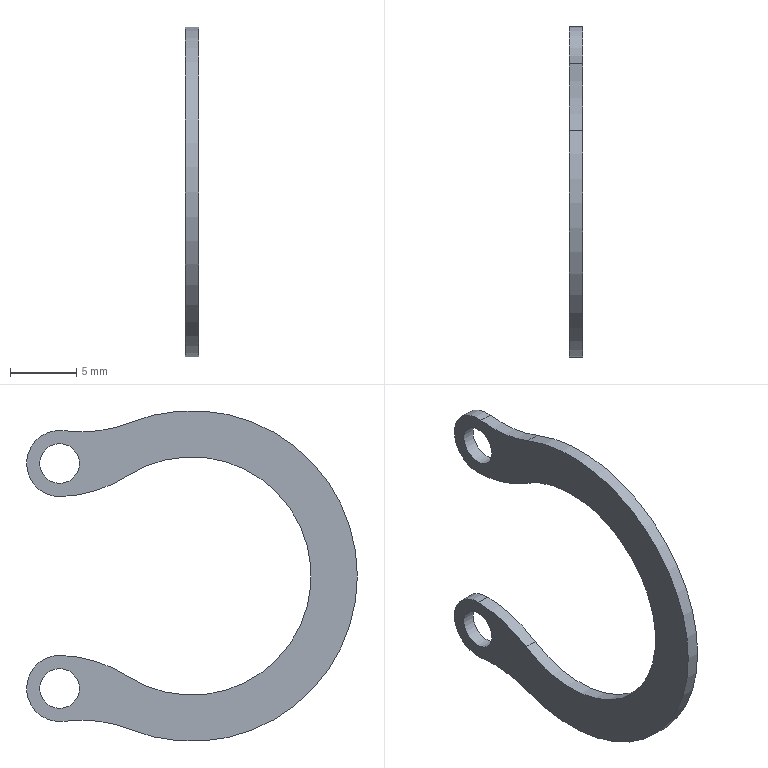Component | NX | SHE_JI-6 | 1 solid | 12 faces | box 1 x 25 x 25 mm | volume 205 mm3 | cylinder 10 | plane 2 | commonest cylinder face diameters 20 x4 5 x2 3 x2 25 x1 18 x1
STEP:
#1=CARTESIAN_POINT('',(0.,0.,0.));
#2=DIRECTION('',(0.,0.,1.));
#3=DIRECTION('',(1.,0.,0.));
#4=AXIS2_PLACEMENT_3D('',#1,#2,#3);
#5=CARTESIAN_POINT('',(85.,29.671,94.022));
#6=VERTEX_POINT('',#5);
#7=CARTESIAN_POINT('',(86.,29.671,94.022));
#8=VERTEX_POINT('',#7);
#9=CARTESIAN_POINT('',(85.,29.671,94.022));
#10=DIRECTION('',(1.,0.,0.));
#11=VECTOR('',#10,1.);
#12=LINE('',#9,#11);
#13=CARTESIAN_POINT('',(85.,28.355,84.109));
#14=DIRECTION('',(1.,0.,0.));
#15=DIRECTION('',(0.,0.,-1.));
#16=AXIS2_PLACEMENT_3D('',#13,#14,#15);
#17=CYLINDRICAL_SURFACE('',#16,10.);
#18=CARTESIAN_POINT('',(3.01,0.));
#19=DIRECTION('',(0.,1.));
#20=VECTOR('',#19,1.);
#21=LINE('',#18,#20);
#22=(GEOMETRIC_REPRESENTATION_CONTEXT(2)PARAMETRIC_REPRESENTATION_CONTEXT()REPRESENTATION_CONTEXT('',''));
#23=DEFINITIONAL_REPRESENTATION('',(#21),#22);
#24=PCURVE('',#17,#23);
#25=CARTESIAN_POINT('',(85.,30.,96.5));
#26=DIRECTION('',(1.,0.,0.));
#27=DIRECTION('',(0.,0.,-1.));
#28=AXIS2_PLACEMENT_3D('',#25,#26,#27);
#29=CYLINDRICAL_SURFACE('',#28,2.5);
#30=CARTESIAN_POINT('',(-0.132,0.));
#31=DIRECTION('',(0.,1.));
#32=VECTOR('',#31,1.);
#33=LINE('',#30,#32);
#34=(GEOMETRIC_REPRESENTATION_CONTEXT(2)PARAMETRIC_REPRESENTATION_CONTEXT()REPRESENTATION_CONTEXT('',''));
#35=DEFINITIONAL_REPRESENTATION('',(#33),#34);
#36=PCURVE('',#29,#35);
#37=SURFACE_CURVE('',#12,(#24,#36),.PCURVE_S1.);
#38=EDGE_CURVE('',#6,#8,#37,.T.);
#39=ORIENTED_EDGE('',*,*,#38,.F.);
#40=CARTESIAN_POINT('',(85.,24.642,93.394));
#41=VERTEX_POINT('',#40);
#42=CARTESIAN_POINT('',(85.,28.355,84.109));
#43=DIRECTION('',(1.,0.,0.));
#44=DIRECTION('',(0.,0.,1.));
#45=AXIS2_PLACEMENT_3D('',#42,#43,#44);
#46=CIRCLE('',#45,10.);
#47=CARTESIAN_POINT('',(-3.142,0.));
#48=DIRECTION('',(1.,0.));
#49=VECTOR('',#48,1.);
#50=LINE('',#47,#49);
#51=(GEOMETRIC_REPRESENTATION_CONTEXT(2)PARAMETRIC_REPRESENTATION_CONTEXT()REPRESENTATION_CONTEXT('',''));
#52=DEFINITIONAL_REPRESENTATION('',(#50),#51);
#53=PCURVE('',#17,#52);
#54=CARTESIAN_POINT('',(85.,24.177,94.554));
#55=DIRECTION('',(1.,0.,0.));
#56=DIRECTION('',(0.,0.,-1.));
#57=AXIS2_PLACEMENT_3D('',#54,#55,#56);
#58=PLANE('',#57);
#59=CARTESIAN_POINT('',(10.446,4.177));
#60=DIRECTION('',(-1.,0.));
#61=AXIS2_PLACEMENT_2D('',#59,#60);
#62=CIRCLE('',#61,10.);
#63=(GEOMETRIC_REPRESENTATION_CONTEXT(2)PARAMETRIC_REPRESENTATION_CONTEXT()REPRESENTATION_CONTEXT('',''));
#64=DEFINITIONAL_REPRESENTATION('',(#62),#63);
#65=PCURVE('',#58,#64);
#66=SURFACE_CURVE('',#46,(#53,#65),.PCURVE_S1.);
#67=EDGE_CURVE('',#6,#41,#66,.T.);
#68=ORIENTED_EDGE('',*,*,#67,.T.);
#69=CARTESIAN_POINT('',(86.,24.642,93.394));
#70=VERTEX_POINT('',#69);
#71=CARTESIAN_POINT('',(85.,24.642,93.394));
#72=DIRECTION('',(1.,0.,0.));
#73=VECTOR('',#72,1.);
#74=LINE('',#71,#73);
#75=CARTESIAN_POINT('',(3.522,0.));
#76=DIRECTION('',(0.,1.));
#77=VECTOR('',#76,1.);
#78=LINE('',#75,#77);
#79=(GEOMETRIC_REPRESENTATION_CONTEXT(2)PARAMETRIC_REPRESENTATION_CONTEXT()REPRESENTATION_CONTEXT('',''));
#80=DEFINITIONAL_REPRESENTATION('',(#78),#79);
#81=PCURVE('',#17,#80);
#82=CARTESIAN_POINT('',(85.,20.,105.));
#83=DIRECTION('',(1.,0.,0.));
#84=DIRECTION('',(0.,0.,-1.));
#85=AXIS2_PLACEMENT_3D('',#82,#83,#84);
#86=CYLINDRICAL_SURFACE('',#85,12.5);
#87=CARTESIAN_POINT('',(6.664,0.));
#88=DIRECTION('',(0.,1.));
#89=VECTOR('',#88,1.);
#90=LINE('',#87,#89);
#91=(GEOMETRIC_REPRESENTATION_CONTEXT(2)PARAMETRIC_REPRESENTATION_CONTEXT()REPRESENTATION_CONTEXT('',''));
#92=DEFINITIONAL_REPRESENTATION('',(#90),#91);
#93=PCURVE('',#86,#92);
#94=SURFACE_CURVE('',#74,(#81,#93),.PCURVE_S1.);
#95=EDGE_CURVE('',#41,#70,#94,.T.);
#96=ORIENTED_EDGE('',*,*,#95,.T.);
#97=CARTESIAN_POINT('',(86.,28.355,84.109));
#98=DIRECTION('',(1.,0.,0.));
#99=DIRECTION('',(0.,0.,1.));
#100=AXIS2_PLACEMENT_3D('',#97,#98,#99);
#101=CIRCLE('',#100,10.);
#102=CARTESIAN_POINT('',(-3.142,1.));
#103=DIRECTION('',(1.,0.));
#104=VECTOR('',#103,1.);
#105=LINE('',#102,#104);
#106=(GEOMETRIC_REPRESENTATION_CONTEXT(2)PARAMETRIC_REPRESENTATION_CONTEXT()REPRESENTATION_CONTEXT('',''));
#107=DEFINITIONAL_REPRESENTATION('',(#105),#106);
#108=PCURVE('',#17,#107);
#109=CARTESIAN_POINT('',(86.,24.177,94.554));
#110=DIRECTION('',(1.,0.,0.));
#111=DIRECTION('',(0.,0.,-1.));
#112=AXIS2_PLACEMENT_3D('',#109,#110,#111);
#113=PLANE('',#112);
#114=CARTESIAN_POINT('',(10.446,4.177));
#115=DIRECTION('',(-1.,0.));
#116=AXIS2_PLACEMENT_2D('',#114,#115);
#117=CIRCLE('',#116,10.);
#118=(GEOMETRIC_REPRESENTATION_CONTEXT(2)PARAMETRIC_REPRESENTATION_CONTEXT()REPRESENTATION_CONTEXT('',''));
#119=DEFINITIONAL_REPRESENTATION('',(#117),#118);
#120=PCURVE('',#113,#119);
#121=SURFACE_CURVE('',#101,(#108,#120),.PCURVE_S1.);
#122=EDGE_CURVE('',#8,#70,#121,.T.);
#123=ORIENTED_EDGE('',*,*,#122,.F.);
#124=EDGE_LOOP('',(#39,#68,#96,#123));
#125=FACE_BOUND('',#124,.F.);
#126=ADVANCED_FACE('',(#125),#17,.F.);
#127=CARTESIAN_POINT('',(86.,24.642,116.606));
#128=VERTEX_POINT('',#127);
#129=CARTESIAN_POINT('',(86.,20.,105.));
#130=DIRECTION('',(-1.,0.,0.));
#131=DIRECTION('',(0.,0.,1.));
#132=AXIS2_PLACEMENT_3D('',#129,#130,#131);
#133=CIRCLE('',#132,12.5);
#134=CARTESIAN_POINT('',(9.425,1.));
#135=DIRECTION('',(-1.,0.));
#136=VECTOR('',#135,1.);
#137=LINE('',#134,#136);
#138=(GEOMETRIC_REPRESENTATION_CONTEXT(2)PARAMETRIC_REPRESENTATION_CONTEXT()REPRESENTATION_CONTEXT('',''));
#139=DEFINITIONAL_REPRESENTATION('',(#137),#138);
#140=PCURVE('',#86,#139);
#141=CARTESIAN_POINT('',(-22.946,-4.177));
#142=CARTESIAN_POINT('',(-22.946,17.473));
#143=CARTESIAN_POINT('',(-4.196,6.648));
#144=CARTESIAN_POINT('',(14.554,-4.177));
#145=CARTESIAN_POINT('',(-4.196,-15.003));
#146=CARTESIAN_POINT('',(-22.946,-25.828));
#147=CARTESIAN_POINT('',(-22.946,-4.177));
#148=(BOUNDED_CURVE()B_SPLINE_CURVE(2,(#141,#142,#143,#144,#145,#146,#147),.UNSPECIFIED.,.T.,.F.)B_SPLINE_CURVE_WITH_KNOTS((1,2,2,2,2,1),(-2.094,0.,2.094,4.189,6.283,8.378),.UNSPECIFIED.)CURVE()GEOMETRIC_REPRESENTATION_ITEM()RATIONAL_B_SPLINE_CURVE((1.,0.5,1.,0.5,1.,0.5,1.))REPRESENTATION_ITEM(''));
#149=(GEOMETRIC_REPRESENTATION_CONTEXT(2)PARAMETRIC_REPRESENTATION_CONTEXT()REPRESENTATION_CONTEXT('',''));
#150=DEFINITIONAL_REPRESENTATION('',(#148),#149);
#151=PCURVE('',#113,#150);
#152=SURFACE_CURVE('',#133,(#140,#151),.PCURVE_S1.);
#153=EDGE_CURVE('',#70,#128,#152,.T.);
#154=ORIENTED_EDGE('',*,*,#153,.T.);
#155=CARTESIAN_POINT('',(85.,24.642,116.606));
#156=VERTEX_POINT('',#155);
#157=CARTESIAN_POINT('',(85.,24.642,116.606));
#158=DIRECTION('',(1.,0.,0.));
#159=VECTOR('',#158,1.);
#160=LINE('',#157,#159);
#161=CARTESIAN_POINT('',(2.761,0.));
#162=DIRECTION('',(0.,1.));
#163=VECTOR('',#162,1.);
#164=LINE('',#161,#163);
#165=(GEOMETRIC_REPRESENTATION_CONTEXT(2)PARAMETRIC_REPRESENTATION_CONTEXT()REPRESENTATION_CONTEXT('',''));
#166=DEFINITIONAL_REPRESENTATION('',(#164),#165);
#167=PCURVE('',#86,#166);
#168=CARTESIAN_POINT('',(85.,28.355,125.891));
#169=DIRECTION('',(1.,0.,0.));
#170=DIRECTION('',(0.,0.,-1.));
#171=AXIS2_PLACEMENT_3D('',#168,#169,#170);
#172=CYLINDRICAL_SURFACE('',#171,10.);
#173=CARTESIAN_POINT('',(5.903,0.));
#174=DIRECTION('',(0.,1.));
#175=VECTOR('',#174,1.);
#176=LINE('',#173,#175);
#177=(GEOMETRIC_REPRESENTATION_CONTEXT(2)PARAMETRIC_REPRESENTATION_CONTEXT()REPRESENTATION_CONTEXT('',''));
#178=DEFINITIONAL_REPRESENTATION('',(#176),#177);
#179=PCURVE('',#172,#178);
#180=SURFACE_CURVE('',#160,(#167,#179),.PCURVE_S1.);
#181=EDGE_CURVE('',#156,#128,#180,.T.);
#182=ORIENTED_EDGE('',*,*,#181,.F.);
#183=CARTESIAN_POINT('',(85.,20.,105.));
#184=DIRECTION('',(-1.,0.,0.));
#185=DIRECTION('',(0.,0.,1.));
#186=AXIS2_PLACEMENT_3D('',#183,#184,#185);
#187=CIRCLE('',#186,12.5);
#188=CARTESIAN_POINT('',(9.425,0.));
#189=DIRECTION('',(-1.,0.));
#190=VECTOR('',#189,1.);
#191=LINE('',#188,#190);
#192=(GEOMETRIC_REPRESENTATION_CONTEXT(2)PARAMETRIC_REPRESENTATION_CONTEXT()REPRESENTATION_CONTEXT('',''));
#193=DEFINITIONAL_REPRESENTATION('',(#191),#192);
#194=PCURVE('',#86,#193);
#195=CARTESIAN_POINT('',(-22.946,-4.177));
#196=CARTESIAN_POINT('',(-22.946,17.473));
#197=CARTESIAN_POINT('',(-4.196,6.648));
#198=CARTESIAN_POINT('',(14.554,-4.177));
#199=CARTESIAN_POINT('',(-4.196,-15.003));
#200=CARTESIAN_POINT('',(-22.946,-25.828));
#201=CARTESIAN_POINT('',(-22.946,-4.177));
#202=(BOUNDED_CURVE()B_SPLINE_CURVE(2,(#195,#196,#197,#198,#199,#200,#201),.UNSPECIFIED.,.T.,.F.)B_SPLINE_CURVE_WITH_KNOTS((1,2,2,2,2,1),(-2.094,0.,2.094,4.189,6.283,8.378),.UNSPECIFIED.)CURVE()GEOMETRIC_REPRESENTATION_ITEM()RATIONAL_B_SPLINE_CURVE((1.,0.5,1.,0.5,1.,0.5,1.))REPRESENTATION_ITEM(''));
#203=(GEOMETRIC_REPRESENTATION_CONTEXT(2)PARAMETRIC_REPRESENTATION_CONTEXT()REPRESENTATION_CONTEXT('',''));
#204=DEFINITIONAL_REPRESENTATION('',(#202),#203);
#205=PCURVE('',#58,#204);
#206=SURFACE_CURVE('',#187,(#194,#205),.PCURVE_S1.);
#207=EDGE_CURVE('',#41,#156,#206,.T.);
#208=ORIENTED_EDGE('',*,*,#207,.F.);
#209=ORIENTED_EDGE('',*,*,#95,.T.);
#210=EDGE_LOOP('',(#154,#182,#208,#209));
#211=FACE_BOUND('',#210,.T.);
#212=ADVANCED_FACE('',(#211),#86,.T.);
#213=ORIENTED_EDGE('',*,*,#181,.F.);
#214=CARTESIAN_POINT('',(85.,29.671,115.978));
#215=VERTEX_POINT('',#214);
#216=CARTESIAN_POINT('',(85.,28.355,125.891));
#217=DIRECTION('',(1.,0.,0.));
#218=DIRECTION('',(0.,0.,-1.));
#219=AXIS2_PLACEMENT_3D('',#216,#217,#218);
#220=CIRCLE('',#219,10.);
#221=CARTESIAN_POINT('',(0.,0.));
#222=DIRECTION('',(1.,0.));
#223=VECTOR('',#222,1.);
#224=LINE('',#221,#223);
#225=(GEOMETRIC_REPRESENTATION_CONTEXT(2)PARAMETRIC_REPRESENTATION_CONTEXT()REPRESENTATION_CONTEXT('',''));
#226=DEFINITIONAL_REPRESENTATION('',(#224),#225);
#227=PCURVE('',#172,#226);
#228=CARTESIAN_POINT('',(-31.337,4.177));
#229=DIRECTION('',(1.,0.));
#230=AXIS2_PLACEMENT_2D('',#228,#229);
#231=CIRCLE('',#230,10.);
#232=(GEOMETRIC_REPRESENTATION_CONTEXT(2)PARAMETRIC_REPRESENTATION_CONTEXT()REPRESENTATION_CONTEXT('',''));
#233=DEFINITIONAL_REPRESENTATION('',(#231),#232);
#234=PCURVE('',#58,#233);
#235=SURFACE_CURVE('',#220,(#227,#234),.PCURVE_S1.);
#236=EDGE_CURVE('',#156,#215,#235,.T.);
#237=ORIENTED_EDGE('',*,*,#236,.T.);
#238=CARTESIAN_POINT('',(86.,29.671,115.978));
#239=VERTEX_POINT('',#238);
#240=CARTESIAN_POINT('',(85.,29.671,115.978));
#241=DIRECTION('',(1.,0.,0.));
#242=VECTOR('',#241,1.);
#243=LINE('',#240,#242);
#244=CARTESIAN_POINT('',(6.415,0.));
#245=DIRECTION('',(0.,1.));
#246=VECTOR('',#245,1.);
#247=LINE('',#244,#246);
#248=(GEOMETRIC_REPRESENTATION_CONTEXT(2)PARAMETRIC_REPRESENTATION_CONTEXT()REPRESENTATION_CONTEXT('',''));
#249=DEFINITIONAL_REPRESENTATION('',(#247),#248);
#250=PCURVE('',#172,#249);
#251=CARTESIAN_POINT('',(85.,30.,113.5));
#252=DIRECTION('',(1.,0.,0.));
#253=DIRECTION('',(0.,0.,-1.));
#254=AXIS2_PLACEMENT_3D('',#251,#252,#253);
#255=CYLINDRICAL_SURFACE('',#254,2.5);
#256=CARTESIAN_POINT('',(3.274,0.));
#257=DIRECTION('',(0.,1.));
#258=VECTOR('',#257,1.);
#259=LINE('',#256,#258);
#260=(GEOMETRIC_REPRESENTATION_CONTEXT(2)PARAMETRIC_REPRESENTATION_CONTEXT()REPRESENTATION_CONTEXT('',''));
#261=DEFINITIONAL_REPRESENTATION('',(#259),#260);
#262=PCURVE('',#255,#261);
#263=SURFACE_CURVE('',#243,(#250,#262),.PCURVE_S1.);
#264=EDGE_CURVE('',#215,#239,#263,.T.);
#265=ORIENTED_EDGE('',*,*,#264,.T.);
#266=CARTESIAN_POINT('',(86.,28.355,125.891));
#267=DIRECTION('',(1.,0.,0.));
#268=DIRECTION('',(0.,0.,-1.));
#269=AXIS2_PLACEMENT_3D('',#266,#267,#268);
#270=CIRCLE('',#269,10.);
#271=CARTESIAN_POINT('',(0.,1.));
#272=DIRECTION('',(1.,0.));
#273=VECTOR('',#272,1.);
#274=LINE('',#271,#273);
#275=(GEOMETRIC_REPRESENTATION_CONTEXT(2)PARAMETRIC_REPRESENTATION_CONTEXT()REPRESENTATION_CONTEXT('',''));
#276=DEFINITIONAL_REPRESENTATION('',(#274),#275);
#277=PCURVE('',#172,#276);
#278=CARTESIAN_POINT('',(-31.337,4.177));
#279=DIRECTION('',(1.,0.));
#280=AXIS2_PLACEMENT_2D('',#278,#279);
#281=CIRCLE('',#280,10.);
#282=(GEOMETRIC_REPRESENTATION_CONTEXT(2)PARAMETRIC_REPRESENTATION_CONTEXT()REPRESENTATION_CONTEXT('',''));
#283=DEFINITIONAL_REPRESENTATION('',(#281),#282);
#284=PCURVE('',#113,#283);
#285=SURFACE_CURVE('',#270,(#277,#284),.PCURVE_S1.);
#286=EDGE_CURVE('',#128,#239,#285,.T.);
#287=ORIENTED_EDGE('',*,*,#286,.F.);
#288=EDGE_LOOP('',(#213,#237,#265,#287));
#289=FACE_BOUND('',#288,.F.);
#290=ADVANCED_FACE('',(#289),#172,.F.);
#291=CARTESIAN_POINT('',(86.,29.915,111.001));
#292=VERTEX_POINT('',#291);
#293=CARTESIAN_POINT('',(86.,30.,113.5));
#294=DIRECTION('',(-1.,0.,0.));
#295=DIRECTION('',(0.,0.,-1.));
#296=AXIS2_PLACEMENT_3D('',#293,#294,#295);
#297=CIRCLE('',#296,2.5);
#298=CARTESIAN_POINT('',(6.283,1.));
#299=DIRECTION('',(-1.,0.));
#300=VECTOR('',#299,1.);
#301=LINE('',#298,#300);
#302=(GEOMETRIC_REPRESENTATION_CONTEXT(2)PARAMETRIC_REPRESENTATION_CONTEXT()REPRESENTATION_CONTEXT('',''));
#303=DEFINITIONAL_REPRESENTATION('',(#301),#302);
#304=PCURVE('',#255,#303);
#305=CARTESIAN_POINT('',(-16.446,5.823));
#306=CARTESIAN_POINT('',(-16.446,1.492));
#307=CARTESIAN_POINT('',(-20.196,3.657));
#308=CARTESIAN_POINT('',(-23.946,5.823));
#309=CARTESIAN_POINT('',(-20.196,7.988));
#310=CARTESIAN_POINT('',(-16.446,10.153));
#311=CARTESIAN_POINT('',(-16.446,5.823));
#312=(BOUNDED_CURVE()B_SPLINE_CURVE(2,(#305,#306,#307,#308,#309,#310,#311),.UNSPECIFIED.,.T.,.F.)B_SPLINE_CURVE_WITH_KNOTS((1,2,2,2,2,1),(-2.094,0.,2.094,4.189,6.283,8.378),.UNSPECIFIED.)CURVE()GEOMETRIC_REPRESENTATION_ITEM()RATIONAL_B_SPLINE_CURVE((1.,0.5,1.,0.5,1.,0.5,1.))REPRESENTATION_ITEM(''));
#313=(GEOMETRIC_REPRESENTATION_CONTEXT(2)PARAMETRIC_REPRESENTATION_CONTEXT()REPRESENTATION_CONTEXT('',''));
#314=DEFINITIONAL_REPRESENTATION('',(#312),#313);
#315=PCURVE('',#113,#314);
#316=SURFACE_CURVE('',#297,(#304,#315),.PCURVE_S1.);
#317=EDGE_CURVE('',#239,#292,#316,.T.);
#318=ORIENTED_EDGE('',*,*,#317,.T.);
#319=CARTESIAN_POINT('',(85.,29.915,111.001));
#320=VERTEX_POINT('',#319);
#321=CARTESIAN_POINT('',(85.,29.915,111.001));
#322=DIRECTION('',(1.,0.,0.));
#323=VECTOR('',#322,1.);
#324=LINE('',#321,#323);
#325=CARTESIAN_POINT('',(-0.03383,0.));
#326=DIRECTION('',(0.,1.));
#327=VECTOR('',#326,1.);
#328=LINE('',#325,#327);
#329=(GEOMETRIC_REPRESENTATION_CONTEXT(2)PARAMETRIC_REPRESENTATION_CONTEXT()REPRESENTATION_CONTEXT('',''));
#330=DEFINITIONAL_REPRESENTATION('',(#328),#329);
#331=PCURVE('',#255,#330);
#332=CARTESIAN_POINT('',(85.,30.254,120.996));
#333=DIRECTION('',(1.,0.,0.));
#334=DIRECTION('',(0.,0.,-1.));
#335=AXIS2_PLACEMENT_3D('',#332,#333,#334);
#336=CYLINDRICAL_SURFACE('',#335,10.);
#337=CARTESIAN_POINT('',(6.249,0.));
#338=DIRECTION('',(0.,1.));
#339=VECTOR('',#338,1.);
#340=LINE('',#337,#339);
#341=(GEOMETRIC_REPRESENTATION_CONTEXT(2)PARAMETRIC_REPRESENTATION_CONTEXT()REPRESENTATION_CONTEXT('',''));
#342=DEFINITIONAL_REPRESENTATION('',(#340),#341);
#343=PCURVE('',#336,#342);
#344=SURFACE_CURVE('',#324,(#331,#343),.PCURVE_S1.);
#345=EDGE_CURVE('',#320,#292,#344,.T.);
#346=ORIENTED_EDGE('',*,*,#345,.F.);
#347=CARTESIAN_POINT('',(85.,30.,113.5));
#348=DIRECTION('',(-1.,0.,0.));
#349=DIRECTION('',(0.,0.,-1.));
#350=AXIS2_PLACEMENT_3D('',#347,#348,#349);
#351=CIRCLE('',#350,2.5);
#352=CARTESIAN_POINT('',(6.283,0.));
#353=DIRECTION('',(-1.,0.));
#354=VECTOR('',#353,1.);
#355=LINE('',#352,#354);
#356=(GEOMETRIC_REPRESENTATION_CONTEXT(2)PARAMETRIC_REPRESENTATION_CONTEXT()REPRESENTATION_CONTEXT('',''));
#357=DEFINITIONAL_REPRESENTATION('',(#355),#356);
#358=PCURVE('',#255,#357);
#359=CARTESIAN_POINT('',(-16.446,5.823));
#360=CARTESIAN_POINT('',(-16.446,1.492));
#361=CARTESIAN_POINT('',(-20.196,3.657));
#362=CARTESIAN_POINT('',(-23.946,5.823));
#363=CARTESIAN_POINT('',(-20.196,7.988));
#364=CARTESIAN_POINT('',(-16.446,10.153));
#365=CARTESIAN_POINT('',(-16.446,5.823));
#366=(BOUNDED_CURVE()B_SPLINE_CURVE(2,(#359,#360,#361,#362,#363,#364,#365),.UNSPECIFIED.,.T.,.F.)B_SPLINE_CURVE_WITH_KNOTS((1,2,2,2,2,1),(-2.094,0.,2.094,4.189,6.283,8.378),.UNSPECIFIED.)CURVE()GEOMETRIC_REPRESENTATION_ITEM()RATIONAL_B_SPLINE_CURVE((1.,0.5,1.,0.5,1.,0.5,1.))REPRESENTATION_ITEM(''));
#367=(GEOMETRIC_REPRESENTATION_CONTEXT(2)PARAMETRIC_REPRESENTATION_CONTEXT()REPRESENTATION_CONTEXT('',''));
#368=DEFINITIONAL_REPRESENTATION('',(#366),#367);
#369=PCURVE('',#58,#368);
#370=SURFACE_CURVE('',#351,(#358,#369),.PCURVE_S1.);
#371=EDGE_CURVE('',#215,#320,#370,.T.);
#372=ORIENTED_EDGE('',*,*,#371,.F.);
#373=ORIENTED_EDGE('',*,*,#264,.T.);
#374=EDGE_LOOP('',(#318,#346,#372,#373));
#375=FACE_BOUND('',#374,.T.);
#376=ADVANCED_FACE('',(#375),#255,.T.);
#377=CARTESIAN_POINT('',(86.,24.857,112.577));
#378=VERTEX_POINT('',#377);
#379=CARTESIAN_POINT('',(86.,30.254,120.996));
#380=DIRECTION('',(-1.,0.,0.));
#381=DIRECTION('',(0.,0.,-1.));
#382=AXIS2_PLACEMENT_3D('',#379,#380,#381);
#383=CIRCLE('',#382,10.);
#384=CARTESIAN_POINT('',(6.283,1.));
#385=DIRECTION('',(-1.,0.));
#386=VECTOR('',#385,1.);
#387=LINE('',#384,#386);
#388=(GEOMETRIC_REPRESENTATION_CONTEXT(2)PARAMETRIC_REPRESENTATION_CONTEXT()REPRESENTATION_CONTEXT('',''));
#389=DEFINITIONAL_REPRESENTATION('',(#387),#388);
#390=PCURVE('',#336,#389);
#391=CARTESIAN_POINT('',(-16.441,6.076));
#392=CARTESIAN_POINT('',(-16.441,-11.244));
#393=CARTESIAN_POINT('',(-31.441,-2.584));
#394=CARTESIAN_POINT('',(-46.441,6.076));
#395=CARTESIAN_POINT('',(-31.441,14.736));
#396=CARTESIAN_POINT('',(-16.441,23.397));
#397=CARTESIAN_POINT('',(-16.441,6.076));
#398=(BOUNDED_CURVE()B_SPLINE_CURVE(2,(#391,#392,#393,#394,#395,#396,#397),.UNSPECIFIED.,.T.,.F.)B_SPLINE_CURVE_WITH_KNOTS((1,2,2,2,2,1),(-2.094,0.,2.094,4.189,6.283,8.378),.UNSPECIFIED.)CURVE()GEOMETRIC_REPRESENTATION_ITEM()RATIONAL_B_SPLINE_CURVE((1.,0.5,1.,0.5,1.,0.5,1.))REPRESENTATION_ITEM(''));
#399=(GEOMETRIC_REPRESENTATION_CONTEXT(2)PARAMETRIC_REPRESENTATION_CONTEXT()REPRESENTATION_CONTEXT('',''));
#400=DEFINITIONAL_REPRESENTATION('',(#398),#399);
#401=PCURVE('',#113,#400);
#402=SURFACE_CURVE('',#383,(#390,#401),.PCURVE_S1.);
#403=EDGE_CURVE('',#292,#378,#402,.T.);
#404=ORIENTED_EDGE('',*,*,#403,.T.);
#405=CARTESIAN_POINT('',(85.,24.857,112.577));
#406=VERTEX_POINT('',#405);
#407=CARTESIAN_POINT('',(85.,24.857,112.577));
#408=DIRECTION('',(1.,0.,0.));
#409=VECTOR('',#408,1.);
#410=LINE('',#407,#409);
#411=CARTESIAN_POINT('',(5.713,0.));
#412=DIRECTION('',(0.,1.));
#413=VECTOR('',#412,1.);
#414=LINE('',#411,#413);
#415=(GEOMETRIC_REPRESENTATION_CONTEXT(2)PARAMETRIC_REPRESENTATION_CONTEXT()REPRESENTATION_CONTEXT('',''));
#416=DEFINITIONAL_REPRESENTATION('',(#414),#415);
#417=PCURVE('',#336,#416);
#418=CARTESIAN_POINT('',(85.,20.,105.));
#419=DIRECTION('',(1.,0.,0.));
#420=DIRECTION('',(0.,0.,-1.));
#421=AXIS2_PLACEMENT_3D('',#418,#419,#420);
#422=CYLINDRICAL_SURFACE('',#421,9.);
#423=CARTESIAN_POINT('',(2.572,0.));
#424=DIRECTION('',(0.,1.));
#425=VECTOR('',#424,1.);
#426=LINE('',#423,#425);
#427=(GEOMETRIC_REPRESENTATION_CONTEXT(2)PARAMETRIC_REPRESENTATION_CONTEXT()REPRESENTATION_CONTEXT('',''));
#428=DEFINITIONAL_REPRESENTATION('',(#426),#427);
#429=PCURVE('',#422,#428);
#430=SURFACE_CURVE('',#410,(#417,#429),.PCURVE_S1.);
#431=EDGE_CURVE('',#406,#378,#430,.T.);
#432=ORIENTED_EDGE('',*,*,#431,.F.);
#433=CARTESIAN_POINT('',(85.,30.254,120.996));
#434=DIRECTION('',(-1.,0.,0.));
#435=DIRECTION('',(0.,0.,-1.));
#436=AXIS2_PLACEMENT_3D('',#433,#434,#435);
#437=CIRCLE('',#436,10.);
#438=CARTESIAN_POINT('',(6.283,0.));
#439=DIRECTION('',(-1.,0.));
#440=VECTOR('',#439,1.);
#441=LINE('',#438,#440);
#442=(GEOMETRIC_REPRESENTATION_CONTEXT(2)PARAMETRIC_REPRESENTATION_CONTEXT()REPRESENTATION_CONTEXT('',''));
#443=DEFINITIONAL_REPRESENTATION('',(#441),#442);
#444=PCURVE('',#336,#443);
#445=CARTESIAN_POINT('',(-16.441,6.076));
#446=CARTESIAN_POINT('',(-16.441,-11.244));
#447=CARTESIAN_POINT('',(-31.441,-2.584));
#448=CARTESIAN_POINT('',(-46.441,6.076));
#449=CARTESIAN_POINT('',(-31.441,14.736));
#450=CARTESIAN_POINT('',(-16.441,23.397));
#451=CARTESIAN_POINT('',(-16.441,6.076));
#452=(BOUNDED_CURVE()B_SPLINE_CURVE(2,(#445,#446,#447,#448,#449,#450,#451),.UNSPECIFIED.,.T.,.F.)B_SPLINE_CURVE_WITH_KNOTS((1,2,2,2,2,1),(-2.094,0.,2.094,4.189,6.283,8.378),.UNSPECIFIED.)CURVE()GEOMETRIC_REPRESENTATION_ITEM()RATIONAL_B_SPLINE_CURVE((1.,0.5,1.,0.5,1.,0.5,1.))REPRESENTATION_ITEM(''));
#453=(GEOMETRIC_REPRESENTATION_CONTEXT(2)PARAMETRIC_REPRESENTATION_CONTEXT()REPRESENTATION_CONTEXT('',''));
#454=DEFINITIONAL_REPRESENTATION('',(#452),#453);
#455=PCURVE('',#58,#454);
#456=SURFACE_CURVE('',#437,(#444,#455),.PCURVE_S1.);
#457=EDGE_CURVE('',#320,#406,#456,.T.);
#458=ORIENTED_EDGE('',*,*,#457,.F.);
#459=ORIENTED_EDGE('',*,*,#345,.T.);
#460=EDGE_LOOP('',(#404,#432,#458,#459));
#461=FACE_BOUND('',#460,.T.);
#462=ADVANCED_FACE('',(#461),#336,.T.);
#463=ORIENTED_EDGE('',*,*,#431,.F.);
#464=CARTESIAN_POINT('',(85.,24.857,97.423));
#465=VERTEX_POINT('',#464);
#466=CARTESIAN_POINT('',(85.,20.,105.));
#467=DIRECTION('',(1.,0.,0.));
#468=DIRECTION('',(0.,0.,1.));
#469=AXIS2_PLACEMENT_3D('',#466,#467,#468);
#470=CIRCLE('',#469,9.);
#471=CARTESIAN_POINT('',(-3.142,0.));
#472=DIRECTION('',(1.,0.));
#473=VECTOR('',#472,1.);
#474=LINE('',#471,#473);
#475=(GEOMETRIC_REPRESENTATION_CONTEXT(2)PARAMETRIC_REPRESENTATION_CONTEXT()REPRESENTATION_CONTEXT('',''));
#476=DEFINITIONAL_REPRESENTATION('',(#474),#475);
#477=PCURVE('',#422,#476);
#478=CARTESIAN_POINT('',(-10.446,-4.177));
#479=DIRECTION('',(-1.,0.));
#480=AXIS2_PLACEMENT_2D('',#478,#479);
#481=CIRCLE('',#480,9.);
#482=(GEOMETRIC_REPRESENTATION_CONTEXT(2)PARAMETRIC_REPRESENTATION_CONTEXT()REPRESENTATION_CONTEXT('',''));
#483=DEFINITIONAL_REPRESENTATION('',(#481),#482);
#484=PCURVE('',#58,#483);
#485=SURFACE_CURVE('',#470,(#477,#484),.PCURVE_S1.);
#486=EDGE_CURVE('',#406,#465,#485,.T.);
#487=ORIENTED_EDGE('',*,*,#486,.T.);
#488=CARTESIAN_POINT('',(86.,24.857,97.423));
#489=VERTEX_POINT('',#488);
#490=CARTESIAN_POINT('',(85.,24.857,97.423));
#491=DIRECTION('',(1.,0.,0.));
#492=VECTOR('',#491,1.);
#493=LINE('',#490,#492);
#494=CARTESIAN_POINT('',(6.853,0.));
#495=DIRECTION('',(0.,1.));
#496=VECTOR('',#495,1.);
#497=LINE('',#494,#496);
#498=(GEOMETRIC_REPRESENTATION_CONTEXT(2)PARAMETRIC_REPRESENTATION_CONTEXT()REPRESENTATION_CONTEXT('',''));
#499=DEFINITIONAL_REPRESENTATION('',(#497),#498);
#500=PCURVE('',#422,#499);
#501=CARTESIAN_POINT('',(85.,30.254,89.004));
#502=DIRECTION('',(1.,0.,0.));
#503=DIRECTION('',(0.,0.,-1.));
#504=AXIS2_PLACEMENT_3D('',#501,#502,#503);
#505=CYLINDRICAL_SURFACE('',#504,10.);
#506=CARTESIAN_POINT('',(3.712,0.));
#507=DIRECTION('',(0.,1.));
#508=VECTOR('',#507,1.);
#509=LINE('',#506,#508);
#510=(GEOMETRIC_REPRESENTATION_CONTEXT(2)PARAMETRIC_REPRESENTATION_CONTEXT()REPRESENTATION_CONTEXT('',''));
#511=DEFINITIONAL_REPRESENTATION('',(#509),#510);
#512=PCURVE('',#505,#511);
#513=SURFACE_CURVE('',#493,(#500,#512),.PCURVE_S1.);
#514=EDGE_CURVE('',#465,#489,#513,.T.);
#515=ORIENTED_EDGE('',*,*,#514,.T.);
#516=CARTESIAN_POINT('',(86.,20.,105.));
#517=DIRECTION('',(1.,0.,0.));
#518=DIRECTION('',(0.,0.,1.));
#519=AXIS2_PLACEMENT_3D('',#516,#517,#518);
#520=CIRCLE('',#519,9.);
#521=CARTESIAN_POINT('',(-3.142,1.));
#522=DIRECTION('',(1.,0.));
#523=VECTOR('',#522,1.);
#524=LINE('',#521,#523);
#525=(GEOMETRIC_REPRESENTATION_CONTEXT(2)PARAMETRIC_REPRESENTATION_CONTEXT()REPRESENTATION_CONTEXT('',''));
#526=DEFINITIONAL_REPRESENTATION('',(#524),#525);
#527=PCURVE('',#422,#526);
#528=CARTESIAN_POINT('',(-10.446,-4.177));
#529=DIRECTION('',(-1.,0.));
#530=AXIS2_PLACEMENT_2D('',#528,#529);
#531=CIRCLE('',#530,9.);
#532=(GEOMETRIC_REPRESENTATION_CONTEXT(2)PARAMETRIC_REPRESENTATION_CONTEXT()REPRESENTATION_CONTEXT('',''));
#533=DEFINITIONAL_REPRESENTATION('',(#531),#532);
#534=PCURVE('',#113,#533);
#535=SURFACE_CURVE('',#520,(#527,#534),.PCURVE_S1.);
#536=EDGE_CURVE('',#378,#489,#535,.T.);
#537=ORIENTED_EDGE('',*,*,#536,.F.);
#538=EDGE_LOOP('',(#463,#487,#515,#537));
#539=FACE_BOUND('',#538,.F.);
#540=ADVANCED_FACE('',(#539),#422,.F.);
#541=CARTESIAN_POINT('',(86.,29.915,98.999));
#542=VERTEX_POINT('',#541);
#543=CARTESIAN_POINT('',(86.,30.254,89.004));
#544=DIRECTION('',(-1.,0.,0.));
#545=DIRECTION('',(0.,0.,1.));
#546=AXIS2_PLACEMENT_3D('',#543,#544,#545);
#547=CIRCLE('',#546,10.);
#548=CARTESIAN_POINT('',(9.425,1.));
#549=DIRECTION('',(-1.,0.));
#550=VECTOR('',#549,1.);
#551=LINE('',#548,#550);
#552=(GEOMETRIC_REPRESENTATION_CONTEXT(2)PARAMETRIC_REPRESENTATION_CONTEXT()REPRESENTATION_CONTEXT('',''));
#553=DEFINITIONAL_REPRESENTATION('',(#551),#552);
#554=PCURVE('',#505,#553);
#555=CARTESIAN_POINT('',(-4.45,6.076));
#556=CARTESIAN_POINT('',(-4.45,23.397));
#557=CARTESIAN_POINT('',(10.55,14.736));
#558=CARTESIAN_POINT('',(25.55,6.076));
#559=CARTESIAN_POINT('',(10.55,-2.584));
#560=CARTESIAN_POINT('',(-4.45,-11.244));
#561=CARTESIAN_POINT('',(-4.45,6.076));
#562=(BOUNDED_CURVE()B_SPLINE_CURVE(2,(#555,#556,#557,#558,#559,#560,#561),.UNSPECIFIED.,.T.,.F.)B_SPLINE_CURVE_WITH_KNOTS((1,2,2,2,2,1),(-2.094,0.,2.094,4.189,6.283,8.378),.UNSPECIFIED.)CURVE()GEOMETRIC_REPRESENTATION_ITEM()RATIONAL_B_SPLINE_CURVE((1.,0.5,1.,0.5,1.,0.5,1.))REPRESENTATION_ITEM(''));
#563=(GEOMETRIC_REPRESENTATION_CONTEXT(2)PARAMETRIC_REPRESENTATION_CONTEXT()REPRESENTATION_CONTEXT('',''));
#564=DEFINITIONAL_REPRESENTATION('',(#562),#563);
#565=PCURVE('',#113,#564);
#566=SURFACE_CURVE('',#547,(#554,#565),.PCURVE_S1.);
#567=EDGE_CURVE('',#489,#542,#566,.T.);
#568=ORIENTED_EDGE('',*,*,#567,.T.);
#569=CARTESIAN_POINT('',(85.,29.915,98.999));
#570=VERTEX_POINT('',#569);
#571=CARTESIAN_POINT('',(85.,29.915,98.999));
#572=DIRECTION('',(1.,0.,0.));
#573=VECTOR('',#572,1.);
#574=LINE('',#571,#573);
#575=CARTESIAN_POINT('',(3.175,0.));
#576=DIRECTION('',(0.,1.));
#577=VECTOR('',#576,1.);
#578=LINE('',#575,#577);
#579=(GEOMETRIC_REPRESENTATION_CONTEXT(2)PARAMETRIC_REPRESENTATION_CONTEXT()REPRESENTATION_CONTEXT('',''));
#580=DEFINITIONAL_REPRESENTATION('',(#578),#579);
#581=PCURVE('',#505,#580);
#582=CARTESIAN_POINT('',(3.175,0.));
#583=DIRECTION('',(0.,1.));
#584=VECTOR('',#583,1.);
#585=LINE('',#582,#584);
#586=(GEOMETRIC_REPRESENTATION_CONTEXT(2)PARAMETRIC_REPRESENTATION_CONTEXT()REPRESENTATION_CONTEXT('',''));
#587=DEFINITIONAL_REPRESENTATION('',(#585),#586);
#588=PCURVE('',#29,#587);
#589=SURFACE_CURVE('',#574,(#581,#588),.PCURVE_S1.);
#590=EDGE_CURVE('',#570,#542,#589,.T.);
#591=ORIENTED_EDGE('',*,*,#590,.F.);
#592=CARTESIAN_POINT('',(85.,30.254,89.004));
#593=DIRECTION('',(-1.,0.,0.));
#594=DIRECTION('',(0.,0.,1.));
#595=AXIS2_PLACEMENT_3D('',#592,#593,#594);
#596=CIRCLE('',#595,10.);
#597=CARTESIAN_POINT('',(9.425,0.));
#598=DIRECTION('',(-1.,0.));
#599=VECTOR('',#598,1.);
#600=LINE('',#597,#599);
#601=(GEOMETRIC_REPRESENTATION_CONTEXT(2)PARAMETRIC_REPRESENTATION_CONTEXT()REPRESENTATION_CONTEXT('',''));
#602=DEFINITIONAL_REPRESENTATION('',(#600),#601);
#603=PCURVE('',#505,#602);
#604=CARTESIAN_POINT('',(-4.45,6.076));
#605=CARTESIAN_POINT('',(-4.45,23.397));
#606=CARTESIAN_POINT('',(10.55,14.736));
#607=CARTESIAN_POINT('',(25.55,6.076));
#608=CARTESIAN_POINT('',(10.55,-2.584));
#609=CARTESIAN_POINT('',(-4.45,-11.244));
#610=CARTESIAN_POINT('',(-4.45,6.076));
#611=(BOUNDED_CURVE()B_SPLINE_CURVE(2,(#604,#605,#606,#607,#608,#609,#610),.UNSPECIFIED.,.T.,.F.)B_SPLINE_CURVE_WITH_KNOTS((1,2,2,2,2,1),(-2.094,0.,2.094,4.189,6.283,8.378),.UNSPECIFIED.)CURVE()GEOMETRIC_REPRESENTATION_ITEM()RATIONAL_B_SPLINE_CURVE((1.,0.5,1.,0.5,1.,0.5,1.))REPRESENTATION_ITEM(''));
#612=(GEOMETRIC_REPRESENTATION_CONTEXT(2)PARAMETRIC_REPRESENTATION_CONTEXT()REPRESENTATION_CONTEXT('',''));
#613=DEFINITIONAL_REPRESENTATION('',(#611),#612);
#614=PCURVE('',#58,#613);
#615=SURFACE_CURVE('',#596,(#603,#614),.PCURVE_S1.);
#616=EDGE_CURVE('',#465,#570,#615,.T.);
#617=ORIENTED_EDGE('',*,*,#616,.F.);
#618=ORIENTED_EDGE('',*,*,#514,.T.);
#619=EDGE_LOOP('',(#568,#591,#617,#618));
#620=FACE_BOUND('',#619,.T.);
#621=ADVANCED_FACE('',(#620),#505,.T.);
#622=CARTESIAN_POINT('',(85.,30.,98.));
#623=VERTEX_POINT('',#622);
#624=CARTESIAN_POINT('',(85.,30.,96.5));
#625=DIRECTION('',(-1.,0.,0.));
#626=DIRECTION('',(0.,0.,1.));
#627=AXIS2_PLACEMENT_3D('',#624,#625,#626);
#628=CIRCLE('',#627,1.5);
#629=CARTESIAN_POINT('',(85.,30.,96.5));
#630=DIRECTION('',(1.,0.,0.));
#631=DIRECTION('',(0.,0.,-1.));
#632=AXIS2_PLACEMENT_3D('',#629,#630,#631);
#633=CYLINDRICAL_SURFACE('',#632,1.5);
#634=CARTESIAN_POINT('',(9.425,0.));
#635=DIRECTION('',(-1.,0.));
#636=VECTOR('',#635,1.);
#637=LINE('',#634,#636);
#638=(GEOMETRIC_REPRESENTATION_CONTEXT(2)PARAMETRIC_REPRESENTATION_CONTEXT()REPRESENTATION_CONTEXT('',''));
#639=DEFINITIONAL_REPRESENTATION('',(#637),#638);
#640=PCURVE('',#633,#639);
#641=CARTESIAN_POINT('',(-3.446,5.823));
#642=CARTESIAN_POINT('',(-3.446,8.421));
#643=CARTESIAN_POINT('',(-1.196,7.122));
#644=CARTESIAN_POINT('',(1.054,5.823));
#645=CARTESIAN_POINT('',(-1.196,4.524));
#646=CARTESIAN_POINT('',(-3.446,3.224));
#647=CARTESIAN_POINT('',(-3.446,5.823));
#648=(BOUNDED_CURVE()B_SPLINE_CURVE(2,(#641,#642,#643,#644,#645,#646,#647),.UNSPECIFIED.,.T.,.F.)B_SPLINE_CURVE_WITH_KNOTS((1,2,2,2,2,1),(-2.094,0.,2.094,4.189,6.283,8.378),.UNSPECIFIED.)CURVE()GEOMETRIC_REPRESENTATION_ITEM()RATIONAL_B_SPLINE_CURVE((1.,0.5,1.,0.5,1.,0.5,1.))REPRESENTATION_ITEM(''));
#649=(GEOMETRIC_REPRESENTATION_CONTEXT(2)PARAMETRIC_REPRESENTATION_CONTEXT()REPRESENTATION_CONTEXT('',''));
#650=DEFINITIONAL_REPRESENTATION('',(#648),#649);
#651=PCURVE('',#58,#650);
#652=SURFACE_CURVE('',#628,(#640,#651),.PCURVE_S1.);
#653=EDGE_CURVE('',#623,#623,#652,.T.);
#654=ORIENTED_EDGE('',*,*,#653,.F.);
#655=CARTESIAN_POINT('',(86.,30.,98.));
#656=VERTEX_POINT('',#655);
#657=CARTESIAN_POINT('',(85.,30.,98.));
#658=CARTESIAN_POINT('',(86.,30.,98.));
#659=B_SPLINE_CURVE_WITH_KNOTS('',1,(#657,#658),.UNSPECIFIED.,.F.,.F.,(2,2),(0.,1.),.PIECEWISE_BEZIER_KNOTS.);
#660=CARTESIAN_POINT('',(9.425,0.));
#661=DIRECTION('',(0.,1.));
#662=VECTOR('',#661,1.);
#663=LINE('',#660,#662);
#664=(GEOMETRIC_REPRESENTATION_CONTEXT(2)PARAMETRIC_REPRESENTATION_CONTEXT()REPRESENTATION_CONTEXT('',''));
#665=DEFINITIONAL_REPRESENTATION('',(#663),#664);
#666=PCURVE('',#633,#665);
#667=CARTESIAN_POINT('',(3.142,0.));
#668=DIRECTION('',(0.,1.));
#669=VECTOR('',#668,1.);
#670=LINE('',#667,#669);
#671=(GEOMETRIC_REPRESENTATION_CONTEXT(2)PARAMETRIC_REPRESENTATION_CONTEXT()REPRESENTATION_CONTEXT('',''));
#672=DEFINITIONAL_REPRESENTATION('',(#670),#671);
#673=PCURVE('',#633,#672);
#674=SEAM_CURVE('',#659,(#666,#673),.PCURVE_S1.);
#675=EDGE_CURVE('',#623,#656,#674,.T.);
#676=ORIENTED_EDGE('',*,*,#675,.T.);
#677=CARTESIAN_POINT('',(86.,30.,96.5));
#678=DIRECTION('',(-1.,0.,0.));
#679=DIRECTION('',(0.,0.,1.));
#680=AXIS2_PLACEMENT_3D('',#677,#678,#679);
#681=CIRCLE('',#680,1.5);
#682=CARTESIAN_POINT('',(9.425,1.));
#683=DIRECTION('',(-1.,0.));
#684=VECTOR('',#683,1.);
#685=LINE('',#682,#684);
#686=(GEOMETRIC_REPRESENTATION_CONTEXT(2)PARAMETRIC_REPRESENTATION_CONTEXT()REPRESENTATION_CONTEXT('',''));
#687=DEFINITIONAL_REPRESENTATION('',(#685),#686);
#688=PCURVE('',#633,#687);
#689=CARTESIAN_POINT('',(-3.446,5.823));
#690=CARTESIAN_POINT('',(-3.446,8.421));
#691=CARTESIAN_POINT('',(-1.196,7.122));
#692=CARTESIAN_POINT('',(1.054,5.823));
#693=CARTESIAN_POINT('',(-1.196,4.524));
#694=CARTESIAN_POINT('',(-3.446,3.224));
#695=CARTESIAN_POINT('',(-3.446,5.823));
#696=(BOUNDED_CURVE()B_SPLINE_CURVE(2,(#689,#690,#691,#692,#693,#694,#695),.UNSPECIFIED.,.T.,.F.)B_SPLINE_CURVE_WITH_KNOTS((1,2,2,2,2,1),(-2.094,0.,2.094,4.189,6.283,8.378),.UNSPECIFIED.)CURVE()GEOMETRIC_REPRESENTATION_ITEM()RATIONAL_B_SPLINE_CURVE((1.,0.5,1.,0.5,1.,0.5,1.))REPRESENTATION_ITEM(''));
#697=(GEOMETRIC_REPRESENTATION_CONTEXT(2)PARAMETRIC_REPRESENTATION_CONTEXT()REPRESENTATION_CONTEXT('',''));
#698=DEFINITIONAL_REPRESENTATION('',(#696),#697);
#699=PCURVE('',#113,#698);
#700=SURFACE_CURVE('',#681,(#688,#699),.PCURVE_S1.);
#701=EDGE_CURVE('',#656,#656,#700,.T.);
#702=ORIENTED_EDGE('',*,*,#701,.T.);
#703=ORIENTED_EDGE('',*,*,#675,.F.);
#704=EDGE_LOOP('',(#654,#676,#702,#703));
#705=FACE_BOUND('',#704,.F.);
#706=ADVANCED_FACE('',(#705),#633,.F.);
#707=CARTESIAN_POINT('',(86.,30.,96.5));
#708=DIRECTION('',(-1.,0.,0.));
#709=DIRECTION('',(0.,0.,1.));
#710=AXIS2_PLACEMENT_3D('',#707,#708,#709);
#711=CIRCLE('',#710,2.5);
#712=CARTESIAN_POINT('',(9.425,1.));
#713=DIRECTION('',(-1.,0.));
#714=VECTOR('',#713,1.);
#715=LINE('',#712,#714);
#716=(GEOMETRIC_REPRESENTATION_CONTEXT(2)PARAMETRIC_REPRESENTATION_CONTEXT()REPRESENTATION_CONTEXT('',''));
#717=DEFINITIONAL_REPRESENTATION('',(#715),#716);
#718=PCURVE('',#29,#717);
#719=CARTESIAN_POINT('',(-4.446,5.823));
#720=CARTESIAN_POINT('',(-4.446,10.153));
#721=CARTESIAN_POINT('',(-0.6956,7.988));
#722=CARTESIAN_POINT('',(3.054,5.823));
#723=CARTESIAN_POINT('',(-0.6956,3.657));
#724=CARTESIAN_POINT('',(-4.446,1.492));
#725=CARTESIAN_POINT('',(-4.446,5.823));
#726=(BOUNDED_CURVE()B_SPLINE_CURVE(2,(#719,#720,#721,#722,#723,#724,#725),.UNSPECIFIED.,.T.,.F.)B_SPLINE_CURVE_WITH_KNOTS((1,2,2,2,2,1),(-2.094,0.,2.094,4.189,6.283,8.378),.UNSPECIFIED.)CURVE()GEOMETRIC_REPRESENTATION_ITEM()RATIONAL_B_SPLINE_CURVE((1.,0.5,1.,0.5,1.,0.5,1.))REPRESENTATION_ITEM(''));
#727=(GEOMETRIC_REPRESENTATION_CONTEXT(2)PARAMETRIC_REPRESENTATION_CONTEXT()REPRESENTATION_CONTEXT('',''));
#728=DEFINITIONAL_REPRESENTATION('',(#726),#727);
#729=PCURVE('',#113,#728);
#730=SURFACE_CURVE('',#711,(#718,#729),.PCURVE_S1.);
#731=EDGE_CURVE('',#542,#8,#730,.T.);
#732=ORIENTED_EDGE('',*,*,#731,.T.);
#733=ORIENTED_EDGE('',*,*,#38,.F.);
#734=CARTESIAN_POINT('',(85.,30.,96.5));
#735=DIRECTION('',(-1.,0.,0.));
#736=DIRECTION('',(0.,0.,1.));
#737=AXIS2_PLACEMENT_3D('',#734,#735,#736);
#738=CIRCLE('',#737,2.5);
#739=CARTESIAN_POINT('',(9.425,0.));
#740=DIRECTION('',(-1.,0.));
#741=VECTOR('',#740,1.);
#742=LINE('',#739,#741);
#743=(GEOMETRIC_REPRESENTATION_CONTEXT(2)PARAMETRIC_REPRESENTATION_CONTEXT()REPRESENTATION_CONTEXT('',''));
#744=DEFINITIONAL_REPRESENTATION('',(#742),#743);
#745=PCURVE('',#29,#744);
#746=CARTESIAN_POINT('',(-4.446,5.823));
#747=CARTESIAN_POINT('',(-4.446,10.153));
#748=CARTESIAN_POINT('',(-0.6956,7.988));
#749=CARTESIAN_POINT('',(3.054,5.823));
#750=CARTESIAN_POINT('',(-0.6956,3.657));
#751=CARTESIAN_POINT('',(-4.446,1.492));
#752=CARTESIAN_POINT('',(-4.446,5.823));
#753=(BOUNDED_CURVE()B_SPLINE_CURVE(2,(#746,#747,#748,#749,#750,#751,#752),.UNSPECIFIED.,.T.,.F.)B_SPLINE_CURVE_WITH_KNOTS((1,2,2,2,2,1),(-2.094,0.,2.094,4.189,6.283,8.378),.UNSPECIFIED.)CURVE()GEOMETRIC_REPRESENTATION_ITEM()RATIONAL_B_SPLINE_CURVE((1.,0.5,1.,0.5,1.,0.5,1.))REPRESENTATION_ITEM(''));
#754=(GEOMETRIC_REPRESENTATION_CONTEXT(2)PARAMETRIC_REPRESENTATION_CONTEXT()REPRESENTATION_CONTEXT('',''));
#755=DEFINITIONAL_REPRESENTATION('',(#753),#754);
#756=PCURVE('',#58,#755);
#757=SURFACE_CURVE('',#738,(#745,#756),.PCURVE_S1.);
#758=EDGE_CURVE('',#570,#6,#757,.T.);
#759=ORIENTED_EDGE('',*,*,#758,.F.);
#760=ORIENTED_EDGE('',*,*,#590,.T.);
#761=EDGE_LOOP('',(#732,#733,#759,#760));
#762=FACE_BOUND('',#761,.T.);
#763=ADVANCED_FACE('',(#762),#29,.T.);
#764=CARTESIAN_POINT('',(85.,30.,115.));
#765=VERTEX_POINT('',#764);
#766=CARTESIAN_POINT('',(85.,30.,113.5));
#767=DIRECTION('',(-1.,0.,0.));
#768=DIRECTION('',(0.,0.,1.));
#769=AXIS2_PLACEMENT_3D('',#766,#767,#768);
#770=CIRCLE('',#769,1.5);
#771=CARTESIAN_POINT('',(85.,30.,113.5));
#772=DIRECTION('',(1.,0.,0.));
#773=DIRECTION('',(0.,0.,-1.));
#774=AXIS2_PLACEMENT_3D('',#771,#772,#773);
#775=CYLINDRICAL_SURFACE('',#774,1.5);
#776=CARTESIAN_POINT('',(9.425,0.));
#777=DIRECTION('',(-1.,0.));
#778=VECTOR('',#777,1.);
#779=LINE('',#776,#778);
#780=(GEOMETRIC_REPRESENTATION_CONTEXT(2)PARAMETRIC_REPRESENTATION_CONTEXT()REPRESENTATION_CONTEXT('',''));
#781=DEFINITIONAL_REPRESENTATION('',(#779),#780);
#782=PCURVE('',#775,#781);
#783=CARTESIAN_POINT('',(-20.446,5.823));
#784=CARTESIAN_POINT('',(-20.446,8.421));
#785=CARTESIAN_POINT('',(-18.196,7.122));
#786=CARTESIAN_POINT('',(-15.946,5.823));
#787=CARTESIAN_POINT('',(-18.196,4.524));
#788=CARTESIAN_POINT('',(-20.446,3.224));
#789=CARTESIAN_POINT('',(-20.446,5.823));
#790=(BOUNDED_CURVE()B_SPLINE_CURVE(2,(#783,#784,#785,#786,#787,#788,#789),.UNSPECIFIED.,.T.,.F.)B_SPLINE_CURVE_WITH_KNOTS((1,2,2,2,2,1),(-2.094,0.,2.094,4.189,6.283,8.378),.UNSPECIFIED.)CURVE()GEOMETRIC_REPRESENTATION_ITEM()RATIONAL_B_SPLINE_CURVE((1.,0.5,1.,0.5,1.,0.5,1.))REPRESENTATION_ITEM(''));
#791=(GEOMETRIC_REPRESENTATION_CONTEXT(2)PARAMETRIC_REPRESENTATION_CONTEXT()REPRESENTATION_CONTEXT('',''));
#792=DEFINITIONAL_REPRESENTATION('',(#790),#791);
#793=PCURVE('',#58,#792);
#794=SURFACE_CURVE('',#770,(#782,#793),.PCURVE_S1.);
#795=EDGE_CURVE('',#765,#765,#794,.T.);
#796=ORIENTED_EDGE('',*,*,#795,.F.);
#797=CARTESIAN_POINT('',(86.,30.,115.));
#798=VERTEX_POINT('',#797);
#799=CARTESIAN_POINT('',(85.,30.,115.));
#800=CARTESIAN_POINT('',(86.,30.,115.));
#801=B_SPLINE_CURVE_WITH_KNOTS('',1,(#799,#800),.UNSPECIFIED.,.F.,.F.,(2,2),(0.,1.),.PIECEWISE_BEZIER_KNOTS.);
#802=CARTESIAN_POINT('',(9.425,0.));
#803=DIRECTION('',(0.,1.));
#804=VECTOR('',#803,1.);
#805=LINE('',#802,#804);
#806=(GEOMETRIC_REPRESENTATION_CONTEXT(2)PARAMETRIC_REPRESENTATION_CONTEXT()REPRESENTATION_CONTEXT('',''));
#807=DEFINITIONAL_REPRESENTATION('',(#805),#806);
#808=PCURVE('',#775,#807);
#809=CARTESIAN_POINT('',(3.142,0.));
#810=DIRECTION('',(0.,1.));
#811=VECTOR('',#810,1.);
#812=LINE('',#809,#811);
#813=(GEOMETRIC_REPRESENTATION_CONTEXT(2)PARAMETRIC_REPRESENTATION_CONTEXT()REPRESENTATION_CONTEXT('',''));
#814=DEFINITIONAL_REPRESENTATION('',(#812),#813);
#815=PCURVE('',#775,#814);
#816=SEAM_CURVE('',#801,(#808,#815),.PCURVE_S1.);
#817=EDGE_CURVE('',#765,#798,#816,.T.);
#818=ORIENTED_EDGE('',*,*,#817,.T.);
#819=CARTESIAN_POINT('',(86.,30.,113.5));
#820=DIRECTION('',(-1.,0.,0.));
#821=DIRECTION('',(0.,0.,1.));
#822=AXIS2_PLACEMENT_3D('',#819,#820,#821);
#823=CIRCLE('',#822,1.5);
#824=CARTESIAN_POINT('',(9.425,1.));
#825=DIRECTION('',(-1.,0.));
#826=VECTOR('',#825,1.);
#827=LINE('',#824,#826);
#828=(GEOMETRIC_REPRESENTATION_CONTEXT(2)PARAMETRIC_REPRESENTATION_CONTEXT()REPRESENTATION_CONTEXT('',''));
#829=DEFINITIONAL_REPRESENTATION('',(#827),#828);
#830=PCURVE('',#775,#829);
#831=CARTESIAN_POINT('',(-20.446,5.823));
#832=CARTESIAN_POINT('',(-20.446,8.421));
#833=CARTESIAN_POINT('',(-18.196,7.122));
#834=CARTESIAN_POINT('',(-15.946,5.823));
#835=CARTESIAN_POINT('',(-18.196,4.524));
#836=CARTESIAN_POINT('',(-20.446,3.224));
#837=CARTESIAN_POINT('',(-20.446,5.823));
#838=(BOUNDED_CURVE()B_SPLINE_CURVE(2,(#831,#832,#833,#834,#835,#836,#837),.UNSPECIFIED.,.T.,.F.)B_SPLINE_CURVE_WITH_KNOTS((1,2,2,2,2,1),(-2.094,0.,2.094,4.189,6.283,8.378),.UNSPECIFIED.)CURVE()GEOMETRIC_REPRESENTATION_ITEM()RATIONAL_B_SPLINE_CURVE((1.,0.5,1.,0.5,1.,0.5,1.))REPRESENTATION_ITEM(''));
#839=(GEOMETRIC_REPRESENTATION_CONTEXT(2)PARAMETRIC_REPRESENTATION_CONTEXT()REPRESENTATION_CONTEXT('',''));
#840=DEFINITIONAL_REPRESENTATION('',(#838),#839);
#841=PCURVE('',#113,#840);
#842=SURFACE_CURVE('',#823,(#830,#841),.PCURVE_S1.);
#843=EDGE_CURVE('',#798,#798,#842,.T.);
#844=ORIENTED_EDGE('',*,*,#843,.T.);
#845=ORIENTED_EDGE('',*,*,#817,.F.);
#846=EDGE_LOOP('',(#796,#818,#844,#845));
#847=FACE_BOUND('',#846,.F.);
#848=ADVANCED_FACE('',(#847),#775,.F.);
#849=ORIENTED_EDGE('',*,*,#67,.T.);
#850=ORIENTED_EDGE('',*,*,#207,.T.);
#851=ORIENTED_EDGE('',*,*,#236,.T.);
#852=ORIENTED_EDGE('',*,*,#371,.T.);
#853=ORIENTED_EDGE('',*,*,#457,.T.);
#854=ORIENTED_EDGE('',*,*,#486,.T.);
#855=ORIENTED_EDGE('',*,*,#616,.T.);
#856=ORIENTED_EDGE('',*,*,#758,.T.);
#857=EDGE_LOOP('',(#849,#850,#851,#852,#853,#854,#855,#856));
#858=FACE_BOUND('',#857,.T.);
#859=ORIENTED_EDGE('',*,*,#653,.F.);
#860=EDGE_LOOP('',(#859));
#861=FACE_BOUND('',#860,.T.);
#862=ORIENTED_EDGE('',*,*,#795,.F.);
#863=EDGE_LOOP('',(#862));
#864=FACE_BOUND('',#863,.T.);
#865=ADVANCED_FACE('',(#858,#861,#864),#58,.F.);
#866=ORIENTED_EDGE('',*,*,#122,.F.);
#867=ORIENTED_EDGE('',*,*,#731,.F.);
#868=ORIENTED_EDGE('',*,*,#567,.F.);
#869=ORIENTED_EDGE('',*,*,#536,.F.);
#870=ORIENTED_EDGE('',*,*,#403,.F.);
#871=ORIENTED_EDGE('',*,*,#317,.F.);
#872=ORIENTED_EDGE('',*,*,#286,.F.);
#873=ORIENTED_EDGE('',*,*,#153,.F.);
#874=EDGE_LOOP('',(#866,#867,#868,#869,#870,#871,#872,#873));
#875=FACE_BOUND('',#874,.T.);
#876=ORIENTED_EDGE('',*,*,#701,.T.);
#877=EDGE_LOOP('',(#876));
#878=FACE_BOUND('',#877,.T.);
#879=ORIENTED_EDGE('',*,*,#843,.T.);
#880=EDGE_LOOP('',(#879));
#881=FACE_BOUND('',#880,.T.);
#882=ADVANCED_FACE('',(#875,#878,#881),#113,.T.);
#883=CLOSED_SHELL('',(#126,#212,#290,#376,#462,#540,#621,#706,#763,#848,#865,#882));
#884=MANIFOLD_SOLID_BREP('',#883);
#885=(LENGTH_UNIT()NAMED_UNIT(*)SI_UNIT(.MILLI.,.METRE.));
#886=UNCERTAINTY_MEASURE_WITH_UNIT(LENGTH_MEASURE(0.000002),#885,'','');
#887=(NAMED_UNIT(*)PLANE_ANGLE_UNIT()SI_UNIT($,.RADIAN.));
#888=(NAMED_UNIT(*)SI_UNIT($,.STERADIAN.)SOLID_ANGLE_UNIT());
#889=(GEOMETRIC_REPRESENTATION_CONTEXT(3)GLOBAL_UNCERTAINTY_ASSIGNED_CONTEXT((#886))GLOBAL_UNIT_ASSIGNED_CONTEXT((#885,#887,#888))REPRESENTATION_CONTEXT('',''));
#890=ADVANCED_BREP_SHAPE_REPRESENTATION('',(#4,#884),#889);